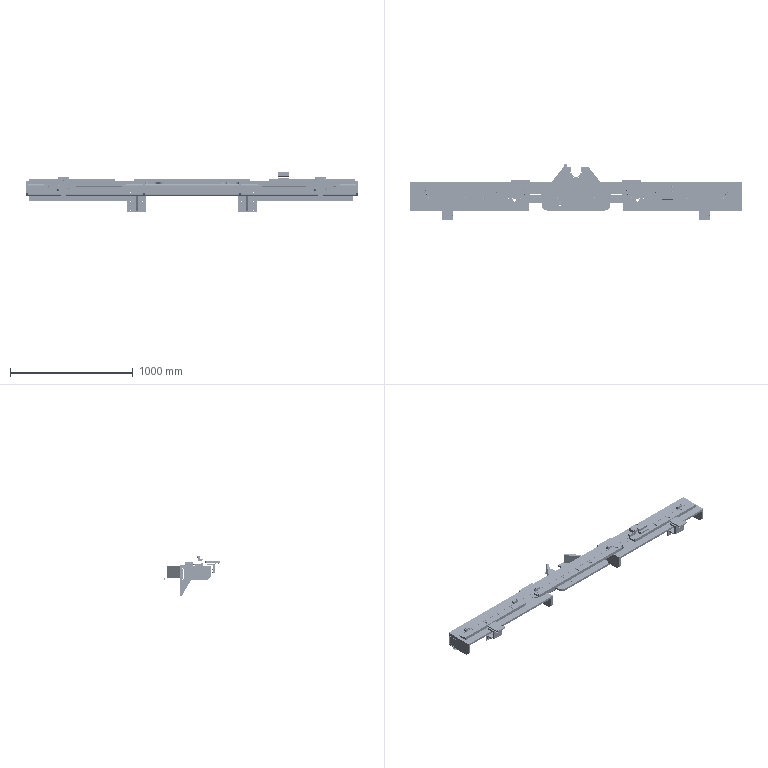Assembly | SolidWorks | mm | 120 component files | 134 solids | 18141 faces | box 2700 x 448 x 328 mm | volume 26324876 mm3 | cone 9802 | cylinder 5951 | plane 2226 | torus 162 | commonest cylinder face diameters 6 x2834 8 x1130 5 x580 10 x404 6.6 x112 9 x103 11 x92 1.2 x72
Bill of materials:
BalanceBlock-0510 | 6 | Q235-A | Rectangular block with two parallel through holes near its ends and one cross hole through the middle of a long side face.
CableChainABracket-0510 | 2 | Q235-A | Thin L-shaped bent bracket: a short flange with two round holes and a long leg with two parallel elongated slots, joined by a radiused bend.
CableChainAGuideSlot-0510 | 2 | Cold Rolled Steel Sheet 08F | Long thin-walled C-shaped channel with unequal flanges and three small holes along one flange.
GuideRailHGL30CA-600 | 2 |  | Long straight bar with a symmetric shaped cross-section (chamfered top corners, small top notches, concave side recesses) and a row of evenly spaced holes through the top face.
HexagonSocketHeadCapScrew-M10X40-0510 | 4 |  | Headed, externally threaded cylindrical fastener shape: a plain cylindrical head with a rounded/chamfered top edge on a straight shank that looks threaded along its full visible length and has a flat end. No drive recess is visible on the head.
HexagonSocketHeadCapScrew-M6X30-0510 | 12 |  | Socket-head cap screw form: cylindrical head with a hex socket, long shank threaded to the end.
HexagonSocketHeadCapScrew-M8X20-0510 | 13 |  | Short socket-head cap screw form: cylindrical head with a hex socket and a threaded shank.
LongFrameSupportA | 1 | Q235-A | Long flat bar with an L-shaped (rabbeted) cross-section and five slotted holes along its length.
ClampingMountingPlateB-0510 | 2 | Q235-A | T-shaped plate with chamfered outer corners, filleted inside corners, a grid of through holes, a thickness step between regions, and small holes in one edge.
FrameLowerPressPlateB-0510 | 2 | Q235-A | Thick rectangular plate with two chamfered corners and eleven through holes in several sizes in a symmetric pattern.
FrictionBlockB-0510 | 2 | Brass | Solid rectangular block with two parallel long top edges rounded by fillets. No holes or other features.
HexagonSocketHeadCapScrew-M6X12-0510 | 8 |  | Short socket-head cap screw form with a hex socket, a short plain neck under the head, and a threaded shank.
HexagonSocketHeadCapScrew-M6X25-0510 | 8 |  | Long socket-head cap screw form, rendered head-down, with a cylindrical head, a short plain neck, and a long threaded shank.
HexagonSocketHeadCapScrew-M8X12-0510 | 16 |  | Short headed fastener-like part: a wide cylindrical head with a short, fully threaded cylindrical shank.
HexSocketHeadCap-M5X45-0510 | 6 |  | Long socket-head cap-screw-like part: a cylindrical head with a hexagonal socket, a long plain shank, and a threaded section toward the tip.
HexSocketHeadCap-M6X16-0510 | 10 |  | Short socket-head cap-screw-like part: a cylindrical head with a hexagonal socket and a fully threaded shank.
LimitB-0510 | 2 | Q235-A | Rectangular U-shaped block: two upright prismatic legs separated by a rectangular slot, joined by a solid base.
PressBlockB-0510 | 2 |  | Rectangular bar/plate with three evenly spaced holes in one long side face and rounded corners on one end.
PullFramePlate-0510 | 2 | Q235-A | Thin flat rectangular plate with two rounded corners at one end and four round through-holes near the opposite end.
LongSideFrameSupportB | 2 | Q235-A | Long slender bar with a stepped (L-shaped) cross-section and four small elongated slots along its length.
LongSideMovingGuideRailBeam-Welded-0510 | 1 | Q235-A | Large, complex elongated beam-like structure: a long flat top plate with downturned end flanges, a widened central section with notches, angled gusset-like plates, and many small holes.
AlignmentStop-0510 | 1 |  | Prismatic stepped block with a Z/L-like profile: a tall upright web with a top overhanging lip, a lower ledge, and chamfered corners.
CylinderConnectionPlate-LongSide-0510 | 1 | Q235-A | Rectangular block with a full-length channel on its underside, giving a bridge-shaped profile, and a pattern of eight holes through the top.
HexagonSocketHeadCapScrew-M6X35-0510 | 4 |  | Socket-head cap-screw-like part of medium length: a cylindrical head with a hexagonal socket, a plain shank section, and a long threaded section.
SensorPlate-0510 | 1 | 304 | Thin sheet-like L-shaped bracket: a long flat flange with two parallel elongated slots, bent at a right angle to a shorter flange.
SliderHGL30CA | 4 |  | Rectangular prismatic block with a full-length U-shaped channel open on the top face. Each channel side wall has two concave rounded grooves running the full length. The top outer edges are chamfered, and the end profile has small notches and chamfers near the base. Small round holes are visible on the end face and near one end of a long side face.
StopA-0510 | 4 | Q235-A | L-shaped bracket of uniform thickness with two legs at roughly a right angle, joined by a rounded outer bend. One leg has two round holes in a line along the part's length. The other leg shows no holes.
Mates:
1. coincident | LongSideMovingGuideRailBeam-Machined-1/LongSideMovingGuideRailBeam-Welded-0510-1 face at (-3425.2, 80.391, 3562.5) dir (0, 0, 1) | RetractableStop-LongSide-1/CylinderConnectionPlate-LongSide-0510-1 face at (-1287.013, 31.236, 3562.5) dir (0, 0, -1)
2. coincident | LongSideMovingGuideRailBeam-Machined-1/LongSideMovingGuideRailBeam-Welded-0510-1 face at (-1721.444, 16.063, 3560.5) dir (0, 0, 1) | LongFrameSupportA-1 face at (-2550.2, -49.609, 3560.5) dir (0, 0, -1)
3. coincident | LongSideMovingGuideRailBeam-Machined-1/LongSideMovingGuideRailBeam-Welded-0510-1 face at (-3425.2, 80.391, 3562.5) dir (0, 0, 1) | BalanceBlock-0510-2 face at (-1407.7, 40.391, 3562.5) dir (0, 0, -1)
4. coincident | LongSideMovingGuideRailBeam-Machined-1/LongSideMovingGuideRailBeam-Welded-0510-1 face at (-3425.2, 80.391, 3562.5) dir (0, 0, 1) | BalanceBlock-0510-4 face at (-2742.7, 40.391, 3562.5) dir (0, 0, -1)
5. concentric | LongSideMovingGuideRailBeam-Machined-1/LongSideMovingGuideRailBeam-Welded-0510-1 face at (-1390.2, 40.391, 3562.5) dir (0, 0, 1) r 3 | BalanceBlock-0510-2 face at (-1390.2, 40.391, 3582.5) dir (0, 0, 1) r 3.3
6. concentric | LongSideMovingGuideRailBeam-Machined-1/LongSideMovingGuideRailBeam-Welded-0510-1 face at (-1425.2, 40.391, 3562.5) dir (0, 0, 1) r 3 | BalanceBlock-0510-2 face at (-1425.2, 40.391, 3582.5) dir (0, 0, 1) r 3.3
7. concentric | LongSideMovingGuideRailBeam-Machined-1/LongSideMovingGuideRailBeam-Welded-0510-1 face at (-2725.2, 40.391, 3562.5) dir (0, 0, 1) r 3 | BalanceBlock-0510-4 face at (-2725.2, 40.391, 3582.5) dir (0, 0, 1) r 3.3
8. concentric | LongSideMovingGuideRailBeam-Machined-1/LongSideMovingGuideRailBeam-Welded-0510-1 face at (-2760.2, 40.391, 3562.5) dir (0, 0, 1) r 3 | BalanceBlock-0510-4 face at (-2760.2, 40.391, 3582.5) dir (0, 0, 1) r 3.3
9. coincident | LongSideMovingGuideRailBeam-Machined-1/LongSideMovingGuideRailBeam-Welded-0510-1 face at (-3425.2, 80.391, 3542.5) dir (0, 0, -1) | GuideRailHGL30CA-600-2 face at (-2645.2, -13.609, 3542.5) dir (0, 0, 1)
10. concentric | LongSideMovingGuideRailBeam-Machined-1/LongSideMovingGuideRailBeam-Welded-0510-1 face at (-3225.2, 0.3914, 3542.5) dir (0, 0, -1) r 3.4 | GuideRailHGL30CA-600-2 face at (-3225.2, 0.3914, 3516.5) dir (0, 0, -1) r 7
11. concentric | LongSideMovingGuideRailBeam-Machined-1/LongSideMovingGuideRailBeam-Welded-0510-1 face at (-3145.2, 0.3914, 3542.5) dir (0, 0, -1) r 3.4 | GuideRailHGL30CA-600-2 face at (-3145.2, 0.3914, 3516.5) dir (0, 0, -1) r 7
12. coincident | GuideRailHGL30CA-600-2 face at (-2645.2, 9.647, 3516.5) dir (0, 0, -1) | SliderHGL30CA-1 face at (-3122.958, 9.647, 3516.5) dir (0, 0, 1)
13. concentric | GuideRailHGL30CA-600-2 face at (-3245.201, -12.335, 3516.983) dir (1, 0, 0) r 2.83 | SliderHGL30CA-1 face at (-3122.958, -12.335, 3516.983) dir (-1, 0, 0) r 2.83
14. coincident | GuideRailHGL30CA-600-2 face at (-2645.2, 9.647, 3516.5) dir (0, 0, -1) | SliderHGL30CA-2 face at (-3020.958, 9.647, 3516.5) dir (0, 0, 1)
15. concentric | GuideRailHGL30CA-600-2 face at (-3245.201, -12.335, 3516.983) dir (1, 0, 0) r 2.83 | SliderHGL30CA-2 face at (-3020.958, -12.335, 3516.983) dir (-1, 0, 0) r 2.83
16. coincident | LongSideMovingGuideRailBeam-Machined-1/LongSideMovingGuideRailBeam-Welded-0510-1 face at (-3425.2, 80.391, 3542.5) dir (0, 0, -1) | assembly face at (-2065.7, -29.109, 3542.5) dir (0, 0, 1)
17. concentric | LongSideMovingGuideRailBeam-Machined-1/LongSideMovingGuideRailBeam-Welded-0510-1 face at (-2092.2, -89.609, 3542.5) dir (0, 0, -1) r 2.1 | assembly face at (-2092.2, -89.609, 3499.7) dir (0, 0, 1) r 2.458
18. concentric | LongSideMovingGuideRailBeam-Machined-1/LongSideMovingGuideRailBeam-Welded-0510-1 face at (-2058.2, -89.609, 3542.5) dir (0, 0, -1) r 2.1 | assembly face at (-2058.2, -89.609, 3499.7) dir (0, 0, 1) r 2.458
19. concentric | SliderHGL30CA-1 face at (-3191.658, -19.609, 3500.5) dir (0, 0, -1) r 4 | LongSideClampingAssemblyBGeneralAssembly-1/ClampingMountingPlateB-0510-1 face at (-3191.658, -19.609, 3486.5) dir (0, 0, -1) r 7.5
20. concentric | SliderHGL30CA-2 face at (-3049.658, 20.391, 3500.5) dir (0, 0, -1) r 4 | LongSideClampingAssemblyBGeneralAssembly-1/ClampingMountingPlateB-0510-1 face at (-3049.658, 20.391, 3486.5) dir (0, 0, -1) r 7.5
21. coincident | SliderHGL30CA-1 face at (-3171.658, 0.3914, 3500.5) dir (0, 0, -1) | LongSideClampingAssemblyBGeneralAssembly-1/ClampingMountingPlateB-0510-1 face at (-3020.658, 35.391, 3500.5) dir (0, 0, 1)
22. coincident | GuideRailHGL30CA-600-3 face at (-1505.2, -8.864, 3516.5) dir (0, 0, -1) | SliderHGL30CA-5 face at (-1032.043, 9.647, 3516.5) dir (0, 0, 1)
23. concentric | GuideRailHGL30CA-600-3 face at (-905.199, -12.335, 3516.983) dir (-1, 0, 0) r 2.83 | SliderHGL30CA-5 face at (-1032.043, -12.335, 3516.983) dir (-1, 0, 0) r 2.83
24. coincident | SliderHGL30CA-5 face at (-1080.743, 0.3914, 3500.5) dir (0, 0, -1) | LongSideClampingAssemblyBGeneralAssembly-2/ClampingMountingPlateB-0510-1 face at (-929.743, 35.391, 3500.5) dir (0, 0, 1)
25. concentric | SliderHGL30CA-5 face at (-1100.743, 20.391, 3500.5) dir (0, 0, -1) r 4 | LongSideClampingAssemblyBGeneralAssembly-2/ClampingMountingPlateB-0510-1 face at (-1100.743, 20.391, 3486.5) dir (0, 0, -1) r 7.5
26. concentric | SliderHGL30CA-4 face at (-998.743, 20.391, 3500.5) dir (0, 0, -1) r 4 | LongSideClampingAssemblyBGeneralAssembly-2/ClampingMountingPlateB-0510-1 face at (-998.743, 20.391, 3486.5) dir (0, 0, -1) r 7.5
27. coincident | LongSideMovingGuideRailBeam-Machined-1/LongSideMovingGuideRailBeam-Welded-0510-1 face at (-1721.444, 16.063, 3560.5) dir (0, 0, 1) | LongSideFrameSupportB-1 face at (-3400.2, -49.609, 3560.5) dir (0, 0, -1)
28. coincident | LongSideMovingGuideRailBeam-Machined-1/LongSideMovingGuideRailBeam-Welded-0510-1 face at (-1721.444, 16.063, 3560.5) dir (0, 0, 1) | LongSideFrameSupportB-2 face at (-1450.2, -49.609, 3560.5) dir (0, 0, -1)
29. coincident | LongSideMovingGuideRailBeam-Machined-1/LongSideMovingGuideRailBeam-Welded-0510-1 face at (-3425.2, 80.391, 3542.5) dir (0, 0, -1) | StopA-0510-1 face at (-905.2, -19.609, 3542.5) dir (0, 0, 1)
30. concentric | LongSideMovingGuideRailBeam-Machined-1/LongSideMovingGuideRailBeam-Welded-0510-1 face at (-885.2, 10.391, 3542.5) dir (0, 0, -1) r 2.5 | StopA-0510-1 face at (-885.2, 10.391, 3537) dir (0, 0, -1) r 3.3
31. concentric | LongSideMovingGuideRailBeam-Machined-1/LongSideMovingGuideRailBeam-Welded-0510-1 face at (-885.2, -9.609, 3542.5) dir (0, 0, -1) r 2.5 | StopA-0510-1 face at (-885.2, -9.609, 3537) dir (0, 0, -1) r 3.3
32. coincident | LongSideMovingGuideRailBeam-Machined-1/LongSideMovingGuideRailBeam-Welded-0510-1 face at (-3425.2, 80.391, 3542.5) dir (0, 0, -1) | StopA-0510-2 face at (-1505.2, 20.391, 3542.5) dir (0, 0, 1)
33. concentric | LongSideMovingGuideRailBeam-Machined-1/LongSideMovingGuideRailBeam-Welded-0510-1 face at (-1525.2, 10.391, 3542.5) dir (0, 0, -1) r 2.5 | StopA-0510-2 face at (-1525.2, 10.391, 3537) dir (0, 0, -1) r 3.3
34. coincident | LongSideMovingGuideRailBeam-Machined-1/LongSideMovingGuideRailBeam-Welded-0510-1 face at (-725.2, 56.391, 3442.5) dir (0, 0, -1) | CableChainAGuideSlot-0510-1 face at (-3400.897, 88.891, 3442.5) dir (0, 0, 1)
35. distance | CableChainAGuideSlot-0510-1 face at (-3400.897, 90.391, 3441) dir (0, 1, 0) | LongSideMovingGuideRailBeam-Machined-1/LongSideMovingGuideRailBeam-Welded-0510-1 face at (-725.2, 120.391, 3526.5) dir (0, 1, 0)
36. coincident | LongSideClampingAssemblyBGeneralAssembly-1/ClampingMountingPlateB-0510-1 face at (-3020.658, 35.391, 3486.5) dir (0, 0, -1) | CableChainABracket-0510-1 face at (-3119.117, -19.609, 3486.5) dir (0, 0, 1)
37. concentric | LongSideClampingAssemblyBGeneralAssembly-1/ClampingMountingPlateB-0510-1 face at (-3131.617, -4.609, 3486.5) dir (0, 0, -1) r 2.5 | CableChainABracket-0510-1 face at (-3131.617, -4.609, 3481.5) dir (0, 0, -1) r 2.75
38. concentric | LongSideClampingAssemblyBGeneralAssembly-1/ClampingMountingPlateB-0510-1 face at (-3106.617, -4.609, 3486.5) dir (0, 0, -1) r 2.5 | CableChainABracket-0510-1 face at (-3106.617, -4.609, 3481.5) dir (0, 0, -1) r 2.75
39. coincident | LongSideMovingGuideRailBeam-Machined-1/LongSideMovingGuideRailBeam-Welded-0510-1 face at (-725.2, 56.391, 3442.5) dir (0, 0, -1) | CableChainAGuideSlot-0510-2 face at (-1565.2, 88.891, 3442.5) dir (0, 0, 1)
40. distance | CableChainAGuideSlot-0510-2 edge at (-765.2, 88.791, 3442.5) dir (0, -1, 0) | LongSideMovingGuideRailBeam-Machined-1/LongSideMovingGuideRailBeam-Welded-0510-1 face at (-725.2, 80.391, 3492.5) dir (1, 0, 0)
41. coincident | CableChainAGuideSlot-0510-1 face at (-3400.897, 88.891, 3441) dir (0, -1, 0) | CableChainAGuideSlot-0510-2 face at (-1565.2, 88.891, 3441) dir (0, -1, 0)
42. coincident | LongSideClampingAssemblyBGeneralAssembly-2/ClampingMountingPlateB-0510-1 face at (-929.743, 35.391, 3486.5) dir (0, 0, -1) | CableChainABracket-0510-2 face at (-1028.201, -19.609, 3486.5) dir (0, 0, 1)
43. concentric | LongSideClampingAssemblyBGeneralAssembly-2/ClampingMountingPlateB-0510-1 face at (-1015.701, -4.609, 3486.5) dir (0, 0, -1) r 2.5 | CableChainABracket-0510-2 face at (-1015.701, -4.609, 3481.5) dir (0, 0, -1) r 2.75
44. concentric | LongSideClampingAssemblyBGeneralAssembly-2/ClampingMountingPlateB-0510-1 face at (-1040.701, -4.609, 3486.5) dir (0, 0, -1) r 2.5 | CableChainABracket-0510-2 face at (-1040.701, -4.609, 3481.5) dir (0, 0, -1) r 2.75
45. concentric | LongSideMovingGuideRailBeam-Machined-1/LongSideMovingGuideRailBeam-Welded-0510-1 face at (-875.2, -9.609, 3560.5) dir (0, 0, 1) r 4 | HexagonSocketHeadCapScrew-M8X20-0510-1 face at (-875.2, -9.609, 3566.5) dir (0, 0, 1) r 6.5
46. coincident | LongSideFrameSupportB-2 face at (-879.7, -15.109, 3566.5) dir (0, 0, 1) | HexagonSocketHeadCapScrew-M8X20-0510-1 face at (-875.2, -9.609, 3566.5) dir (0, 0, -1)
47. coincident | LongSideMovingGuideRailBeam-Machined-1/LongSideMovingGuideRailBeam-Welded-0510-1 face at (-3425.2, 80.391, 3562.5) dir (0, 0, 1) | BalanceBlock-0510-5 face at (-857.7, 40.391, 3562.5) dir (0, 0, -1)
48. concentric | LongSideMovingGuideRailBeam-Machined-1/LongSideMovingGuideRailBeam-Welded-0510-1 face at (-875.2, 40.391, 3562.5) dir (0, 0, 1) r 3 | BalanceBlock-0510-5 face at (-875.2, 40.391, 3582.5) dir (0, 0, 1) r 3.3
49. concentric | LongSideMovingGuideRailBeam-Machined-1/LongSideMovingGuideRailBeam-Welded-0510-1 face at (-840.2, 40.391, 3562.5) dir (0, 0, 1) r 3 | BalanceBlock-0510-5 face at (-840.2, 40.391, 3582.5) dir (0, 0, 1) r 3.3
50. coincident | LongSideMovingGuideRailBeam-Machined-1/LongSideMovingGuideRailBeam-Welded-0510-1 face at (-3425.2, 80.391, 3562.5) dir (0, 0, 1) | BalanceBlock-0510-6 face at (-1657.7, 40.391, 3562.5) dir (0, 0, -1)
51. concentric | LongSideMovingGuideRailBeam-Machined-1/LongSideMovingGuideRailBeam-Welded-0510-1 face at (-1640.2, 40.391, 3562.5) dir (0, 0, 1) r 3 | BalanceBlock-0510-6 face at (-1640.2, 40.391, 3582.5) dir (0, 0, 1) r 3.3
52. concentric | LongSideMovingGuideRailBeam-Machined-1/LongSideMovingGuideRailBeam-Welded-0510-1 face at (-1675.2, 40.391, 3562.5) dir (0, 0, 1) r 3 | BalanceBlock-0510-6 face at (-1675.2, 40.391, 3582.5) dir (0, 0, 1) r 3.3
53. concentric | BalanceBlock-0510-5 face at (-840.2, 40.391, 3582.5) dir (0, 0, 1) r 3.3 | HexagonSocketHeadCapScrew-M6X30-0510-1 face at (-840.2, 40.391, 3545.7) dir (0, 0, 1) r 3
54. coincident | BalanceBlock-0510-5 face at (-836.9, 40.391, 3575.7) dir (0, 0, 1) | HexagonSocketHeadCapScrew-M6X30-0510-1 face at (-840.2, 40.391, 3575.7) dir (0, 0, -1)
55. concentric | BalanceBlock-0510-5 face at (-875.2, 40.391, 3582.5) dir (0, 0, 1) r 3.3 | HexagonSocketHeadCapScrew-M6X30-0510-2 face at (-875.2, 40.391, 3545.7) dir (0, 0, 1) r 3
56. coincident | BalanceBlock-0510-5 face at (-871.9, 40.391, 3575.7) dir (0, 0, 1) | HexagonSocketHeadCapScrew-M6X30-0510-2 face at (-875.2, 40.391, 3575.7) dir (0, 0, -1)
57. concentric | BalanceBlock-0510-2 face at (-1390.2, 40.391, 3582.5) dir (0, 0, 1) r 5.5 | HexagonSocketHeadCapScrew-M6X30-0510-3 face at (-1390.2, 40.391, 3545.7) dir (0, 0, 1) r 3
58. coincident | BalanceBlock-0510-2 face at (-1386.9, 40.391, 3575.7) dir (0, 0, 1) | HexagonSocketHeadCapScrew-M6X30-0510-3 face at (-1390.2, 40.391, 3575.7) dir (0, 0, -1)
59. concentric | BalanceBlock-0510-2 face at (-1425.2, 40.391, 3582.5) dir (0, 0, 1) r 5.5 | HexagonSocketHeadCapScrew-M6X30-0510-4 face at (-1425.2, 40.391, 3545.7) dir (0, 0, 1) r 3
60. coincident | BalanceBlock-0510-2 face at (-1421.9, 40.391, 3575.7) dir (0, 0, 1) | HexagonSocketHeadCapScrew-M6X30-0510-4 face at (-1425.2, 40.391, 3575.7) dir (0, 0, -1)
61. concentric | BalanceBlock-0510-6 face at (-1640.2, 40.391, 3582.5) dir (0, 0, 1) r 3.3 | HexagonSocketHeadCapScrew-M6X30-0510-5 face at (-1640.2, 40.391, 3545.7) dir (0, 0, 1) r 3
62. coincident | BalanceBlock-0510-6 face at (-1636.9, 40.391, 3575.7) dir (0, 0, 1) | HexagonSocketHeadCapScrew-M6X30-0510-5 face at (-1640.2, 40.391, 3575.7) dir (0, 0, -1)
63. concentric | BalanceBlock-0510-6 face at (-1675.2, 40.391, 3582.5) dir (0, 0, 1) r 5.5 | HexagonSocketHeadCapScrew-M6X30-0510-6 face at (-1675.2, 40.391, 3545.7) dir (0, 0, 1) r 3
64. coincident | BalanceBlock-0510-6 face at (-1671.9, 40.391, 3575.7) dir (0, 0, 1) | HexagonSocketHeadCapScrew-M6X30-0510-6 face at (-1675.2, 40.391, 3575.7) dir (0, 0, -1)
65. concentric | BalanceBlock-0510-6 face at (-1657.7, 50.391, 3572.5) dir (0, 1, 0) r 5 | HexagonSocketHeadCapScrew-M10X40-0510-1 face at (-1657.7, 15.391, 3572.5) dir (0, 1, 0) r 5
66. coincident | BalanceBlock-0510-6 face at (-1682.7, 50.391, 3582.5) dir (0, 1, 0) | HexagonSocketHeadCapScrew-M10X40-0510-1 face at (-1657.7, 50.391, 3572.5) dir (0, -1, 0)
67. concentric | BalanceBlock-0510-5 face at (-857.7, 50.391, 3572.5) dir (0, 1, 0) r 5 | HexagonSocketHeadCapScrew-M10X40-0510-3 face at (-857.7, 15.391, 3572.5) dir (0, 1, 0) r 5
68. coincident | BalanceBlock-0510-5 face at (-882.7, 50.391, 3582.5) dir (0, 1, 0) | HexagonSocketHeadCapScrew-M10X40-0510-3 face at (-857.7, 50.391, 3572.5) dir (0, -1, 0)
69. coincident | LongSideMovingGuideRailBeam-Machined-1/LongSideMovingGuideRailBeam-Welded-0510-1 face at (-1721.444, 16.063, 3462.5) dir (0, 0, -1) | SensorPlate-0510-1 face at (-2175.2, 265.391, 3462.5) dir (0, 0, 1)
70. parallel | LongSideMovingGuideRailBeam-Machined-1/LongSideMovingGuideRailBeam-Welded-0510-1 face at (-1975.2, 245.391, 3480.5) dir (0, 1, 0) | SensorPlate-0510-1 face at (-2175.2, 265.391, 3442.5) dir (0, 1, 0)
71. distance | SensorPlate-0510-1 face at (-2175.2, 265.391, 3442.5) dir (0, 1, 0) | LongSideMovingGuideRailBeam-Machined-1/LongSideMovingGuideRailBeam-Welded-0510-1 face at (-1975.2, 245.391, 3480.5) dir (0, 1, 0)
72. coincident | LongSideMovingGuideRailBeam-Machined-1/LongSideMovingGuideRailBeam-Welded-0510-1 vertex at (-2175.2, 245.391, 3462.5) dir (1, 0, 0) | SensorPlate-0510-1 face at (-2175.2, 263.891, 3460.263) dir (-1, 0, 0)
73. slot | LongSideMovingGuideRailBeam-Machined-1/LongSideMovingGuideRailBeam-Welded-0510-1 face at (-2075.2, -9.609, 3560.5) dir (0, 0, 1) r 4 | LongFrameSupportA-1 face at (-2067.7, -4.109, 3575.5) dir (-1, 0, 0)
74. slot | LongSideMovingGuideRailBeam-Machined-1/LongSideMovingGuideRailBeam-Welded-0510-1 face at (-1325.2, -9.609, 3560.5) dir (0, 0, 1) r 4 | LongSideFrameSupportB-2 face at (-1332.7, -4.109, 3566.5) dir (1, 0, 0)
75. slot | LongSideMovingGuideRailBeam-Machined-1/LongSideMovingGuideRailBeam-Welded-0510-1 face at (-2825.2, -9.609, 3560.5) dir (0, 0, 1) r 4 | LongSideFrameSupportB-1 face at (-2825.2, -4.109, 3575.5) dir (0, 0, 1) r 4.5
76. slot | LongSideMovingGuideRailBeam-Machined-1/LongSideMovingGuideRailBeam-Welded-0510-1 face at (-3275.2, -9.609, 3560.5) dir (0, 0, 1) r 4 | LongSideFrameSupportB-1 face at (-3267.7, -4.109, 3575.5) dir (-1, 0, 0)
77. coincident | FrameClampingAssemblyA face at (0, -17.5, 0) dir (-1, 0, 0) | FrameClampingAssemblyA plane at (0, 0, 0) dir (1, 0, 0)
78. coincident | FrameClampingAssemblyA face at (2.3, 0, 0) dir (0, 1, 0) | FrameClampingAssemblyA plane at (0, 0, 0) dir (0, 1, 0)
79. coincident | FrameClampingAssemblyA face at (2.8, -74.4, 0) dir (0, 0, -1) | FrameClampingAssemblyA plane at (0, 0, 0) dir (0, 0, 1)
80. coincident | ClampingMountingPlateB-0510-1 face at (0, 0, 0) dir (0, 0, -1) | LongSideClampingAssemblyBGeneralAssembly plane at (0, 0, 0) dir (0, 0, 1)
81. coincident | ClampingMountingPlateB-0510-1 face at (0, 0, 0) dir (0, -1, 0) | LongSideClampingAssemblyBGeneralAssembly plane at (0, 0, 0) dir (0, 1, 0)
82. coincident | ClampingMountingPlateB-0510-1 face at (0, 0, 0) dir (1, 0, 0) | LongSideClampingAssemblyBGeneralAssembly plane at (0, 0, 0) dir (1, 0, 0)
83. coincident | ClampingMountingPlateB-0510-1 face at (0, 11, 0) dir (0, 1, 0) | LongSideClampingAssemblyBGeneralAssembly face at (-109.5, 11, 69.5) dir (0, -1, 0)
84. coincident | FrameLowerPressPlateB-0510-1 face at (-52.5, 11, 163) dir (0, 0, -1) | LongSideClampingAssemblyBGeneralAssembly face at (-100, 32, 163) dir (0, 0, 1)
85. concentric | ClampingMountingPlateB-0510-1 face at (-83, 0, 130) dir (0, -1, 0) r 5.5 | LongSideClampingAssemblyBGeneralAssembly face at (-83, 53.8, 130) dir (0, -1, 0) r 4.75
86. concentric | ClampingMountingPlateB-0510-1 face at (-117, 0, 130) dir (0, -1, 0) r 5.5 | LongSideClampingAssemblyBGeneralAssembly face at (-117, 53.8, 130) dir (0, -1, 0) r 2.75
87. concentric | FrameLowerPressPlateB-0510-1 face at (-61, 19, 178) dir (0, 0, 1) r 3.3 | LongSideClampingAssemblyBGeneralAssembly face at (-61, 19, 153) dir (0, 0, 1) r 2.458
88. concentric | FrameLowerPressPlateB-0510-1 face at (-139, 19, 178) dir (0, 0, 1) r 3.3 | LongSideClampingAssemblyBGeneralAssembly face at (-139, 19, 153) dir (0, 0, 1) r 2.458
89. coincident | PressBlockB-0510-1 face at (-52.5, 91, 163) dir (0, 0, 1) | FrameLowerPressPlateB-0510-1 face at (-52.5, 11, 163) dir (0, 0, -1)
90. concentric | PressBlockB-0510-1 face at (-70, 83.5, 163) dir (0, 0, 1) r 2.5 | FrameLowerPressPlateB-0510-1 face at (-70, 83.5, 178) dir (0, 0, 1) r 5
91. concentric | PressBlockB-0510-1 face at (-130, 83.5, 163) dir (0, 0, 1) r 2.5 | FrameLowerPressPlateB-0510-1 face at (-130, 83.5, 178) dir (0, 0, 1) r 2.75
92. concentric | ClampingMountingPlateB-0510-1 face at (-83, 0, 130) dir (0, -1, 0) r 3.3 | HexagonSocketHeadCapScrew-M6X25-0510-1 face at (-83, 31.8, 130) dir (0, -1, 0) r 3
93. coincident | ClampingMountingPlateB-0510-1 face at (-83, 6.8, 126.7) dir (0, -1, 0) | HexagonSocketHeadCapScrew-M6X25-0510-1 face at (-83, 6.8, 130) dir (0, 1, 0)
94. coincident | ClampingMountingPlateB-0510-1 face at (-171, 9, 50.5) dir (0, -1, 0) | HexagonSocketHeadCapScrew-M8X12-0510-1 face at (-171, 9, 55) dir (0, 1, 0)
95. concentric | ClampingMountingPlateB-0510-1 face at (-171, 0, 55) dir (0, -1, 0) r 4.5 | HexagonSocketHeadCapScrew-M8X12-0510-1 face at (-171, 9, 55) dir (0, -1, 0) r 6.5
96. coincident | FrameLowerPressPlateB-0510-1 face at (-135.7, 19, 171.2) dir (0, 0, 1) | HexSocketHeadCap-M6X16-0510-1 face at (-139, 19, 171.2) dir (0, 0, -1)
97. concentric | FrameLowerPressPlateB-0510-1 face at (-139, 19, 178) dir (0, 0, 1) r 5.5 | HexSocketHeadCap-M6X16-0510-1 face at (-139, 19, 171.2) dir (0, 0, 1) r 5
98. concentric | PullFramePlate-0510-1 face at (-61, 109, 212) dir (0, 1, 0) r 3.3 | HexagonSocketHeadCapScrew-M6X12-0510-1 face at (-61, 90.2, 212) dir (0, 1, 0) r 3
99. coincident | PullFramePlate-0510-1 face at (-64.3, 102.2, 212) dir (0, 1, 0) | HexagonSocketHeadCapScrew-M6X12-0510-1 face at (-61, 102.2, 212) dir (0, -1, 0)
100. concentric | FrameLowerPressPlateB-0510-1 face at (-70, 83.5, 178) dir (0, 0, 1) r 2.75 | HexSocketHeadCap-M5X45-0510-1 face at (-70, 83.5, 127.3) dir (0, 0, 1) r 2.5
101. coincident | FrameLowerPressPlateB-0510-1 face at (-67.25, 83.5, 172.3) dir (0, 0, 1) | HexSocketHeadCap-M5X45-0510-1 face at (-70, 83.5, 172.3) dir (0, 0, -1)
102. coincident | ClampingMountingPlateB-0510-1 face at (-200, 0, 0) dir (-1, 0, 0) | LimitB-0510-1 face at (-200, 24.5, 35) dir (1, 0, 0)
103. concentric | ClampingMountingPlateB-0510-1 face at (-200, 7, 50) dir (-1, 0, 0) r 2.1 | LimitB-0510-1 face at (-220, 7, 50) dir (-1, 0, 0) r 5
104. concentric | ClampingMountingPlateB-0510-1 face at (-200, 7, 20) dir (-1, 0, 0) r 2.1 | LimitB-0510-1 face at (-220, 7, 20) dir (-1, 0, 0) r 2.75
105. coincident | LimitB-0510-1 face at (-220, 14.5, 50) dir (0, 1, 0) | FrictionBlockB-0510-1 face at (-210, 14.5, 35) dir (0, -1, 0)
106. concentric | LimitB-0510-1 face at (-210, -0.5, 35) dir (0, -1, 0) r 2.5 | FrictionBlockB-0510-1 face at (-210, 14.5, 35) dir (0, -1, 0) r 3.3
107. coincident | LimitB-0510-1 face at (-220, 24.5, 35) dir (-1, 0, 0) | FrictionBlockB-0510-1 face at (-220, 14.5, 50) dir (-1, 0, 0)
108. coincident | CylinderConnectionPlate-LongSide-0510-1 face at (0, 0, 0) dir (0, 0, 1) | RetractableStop-LongSide plane at (0, 0, 0) dir (0, 0, 1)
109. coincident | CylinderConnectionPlate-LongSide-0510-1 face at (0, 0, 0) dir (0, -1, 0) | RetractableStop-LongSide plane at (0, 0, 0) dir (0, 1, 0)
110. coincident | CylinderConnectionPlate-LongSide-0510-1 face at (0, 0, 0) dir (-1, 0, 0) | RetractableStop-LongSide plane at (0, 0, 0) dir (1, 0, 0)
111. concentric | AlignmentStop-0510-1 face at (-53, 64, -6) dir (-1, 0, 0) r 5.5 | HexSocketHeadCap-M6X16-0510-1 face at (-46.2, 64, -6) dir (-1, 0, 0) r 5
112. coincident | AlignmentStop-0510-1 face at (-46.2, 64, -2.7) dir (-1, 0, 0) | HexSocketHeadCap-M6X16-0510-1 face at (-46.2, 64, -6) dir (1, 0, 0)
113. concentric | AlignmentStop-0510-1 face at (-53, 64, -84) dir (-1, 0, 0) r 5.5 | HexSocketHeadCap-M6X16-0510-3 face at (-46.2, 64, -84) dir (-1, 0, 0) r 5
114. concentric | CylinderConnectionPlate-LongSide-0510-1 face at (12.5, 30, -82.5) dir (0, 1, 0) r 3.3 | HexagonSocketHeadCapScrew-M6X35-0510-1 face at (12.5, -25, -82.5) dir (0, 1, 0) r 3
115. coincident | CylinderConnectionPlate-LongSide-0510-1 face at (12.5, 10, -85.8) dir (0, 1, 0) | HexagonSocketHeadCapScrew-M6X35-0510-1 face at (12.5, 10, -82.5) dir (0, -1, 0)
116. concentric | CylinderConnectionPlate-LongSide-0510-1 face at (52.5, 30, -82.5) dir (0, 1, 0) r 3.3 | HexagonSocketHeadCapScrew-M6X35-0510-2 face at (52.5, -25, -82.5) dir (0, 1, 0) r 3
117. coincident | CylinderConnectionPlate-LongSide-0510-1 face at (52.5, 10, -85.8) dir (0, 1, 0) | HexagonSocketHeadCapScrew-M6X35-0510-2 face at (52.5, 10, -82.5) dir (0, -1, 0)
118. concentric | CylinderConnectionPlate-LongSide-0510-1 face at (52.5, 30, -7.5) dir (0, 1, 0) r 3.3 | HexagonSocketHeadCapScrew-M6X35-0510-3 face at (52.5, -25, -7.5) dir (0, 1, 0) r 3
119. coincident | CylinderConnectionPlate-LongSide-0510-1 face at (52.5, 10, -10.8) dir (0, 1, 0) | HexagonSocketHeadCapScrew-M6X35-0510-3 face at (52.5, 10, -7.5) dir (0, -1, 0)
120. concentric | CylinderConnectionPlate-LongSide-0510-1 face at (12.5, 30, -7.5) dir (0, 1, 0) r 3.3 | HexagonSocketHeadCapScrew-M6X35-0510-4 face at (12.5, -25, -7.5) dir (0, 1, 0) r 3
121. coincident | CylinderConnectionPlate-LongSide-0510-1 face at (12.5, 10, -10.8) dir (0, 1, 0) | HexagonSocketHeadCapScrew-M6X35-0510-4 face at (12.5, 10, -7.5) dir (0, -1, 0)
122. coincident | AlignmentStop-0510-1 face at (-46.2, 64, -80.7) dir (-1, 0, 0) | HexSocketHeadCap-M6X16-0510-3 face at (-46.2, 64, -84) dir (1, 0, 0)